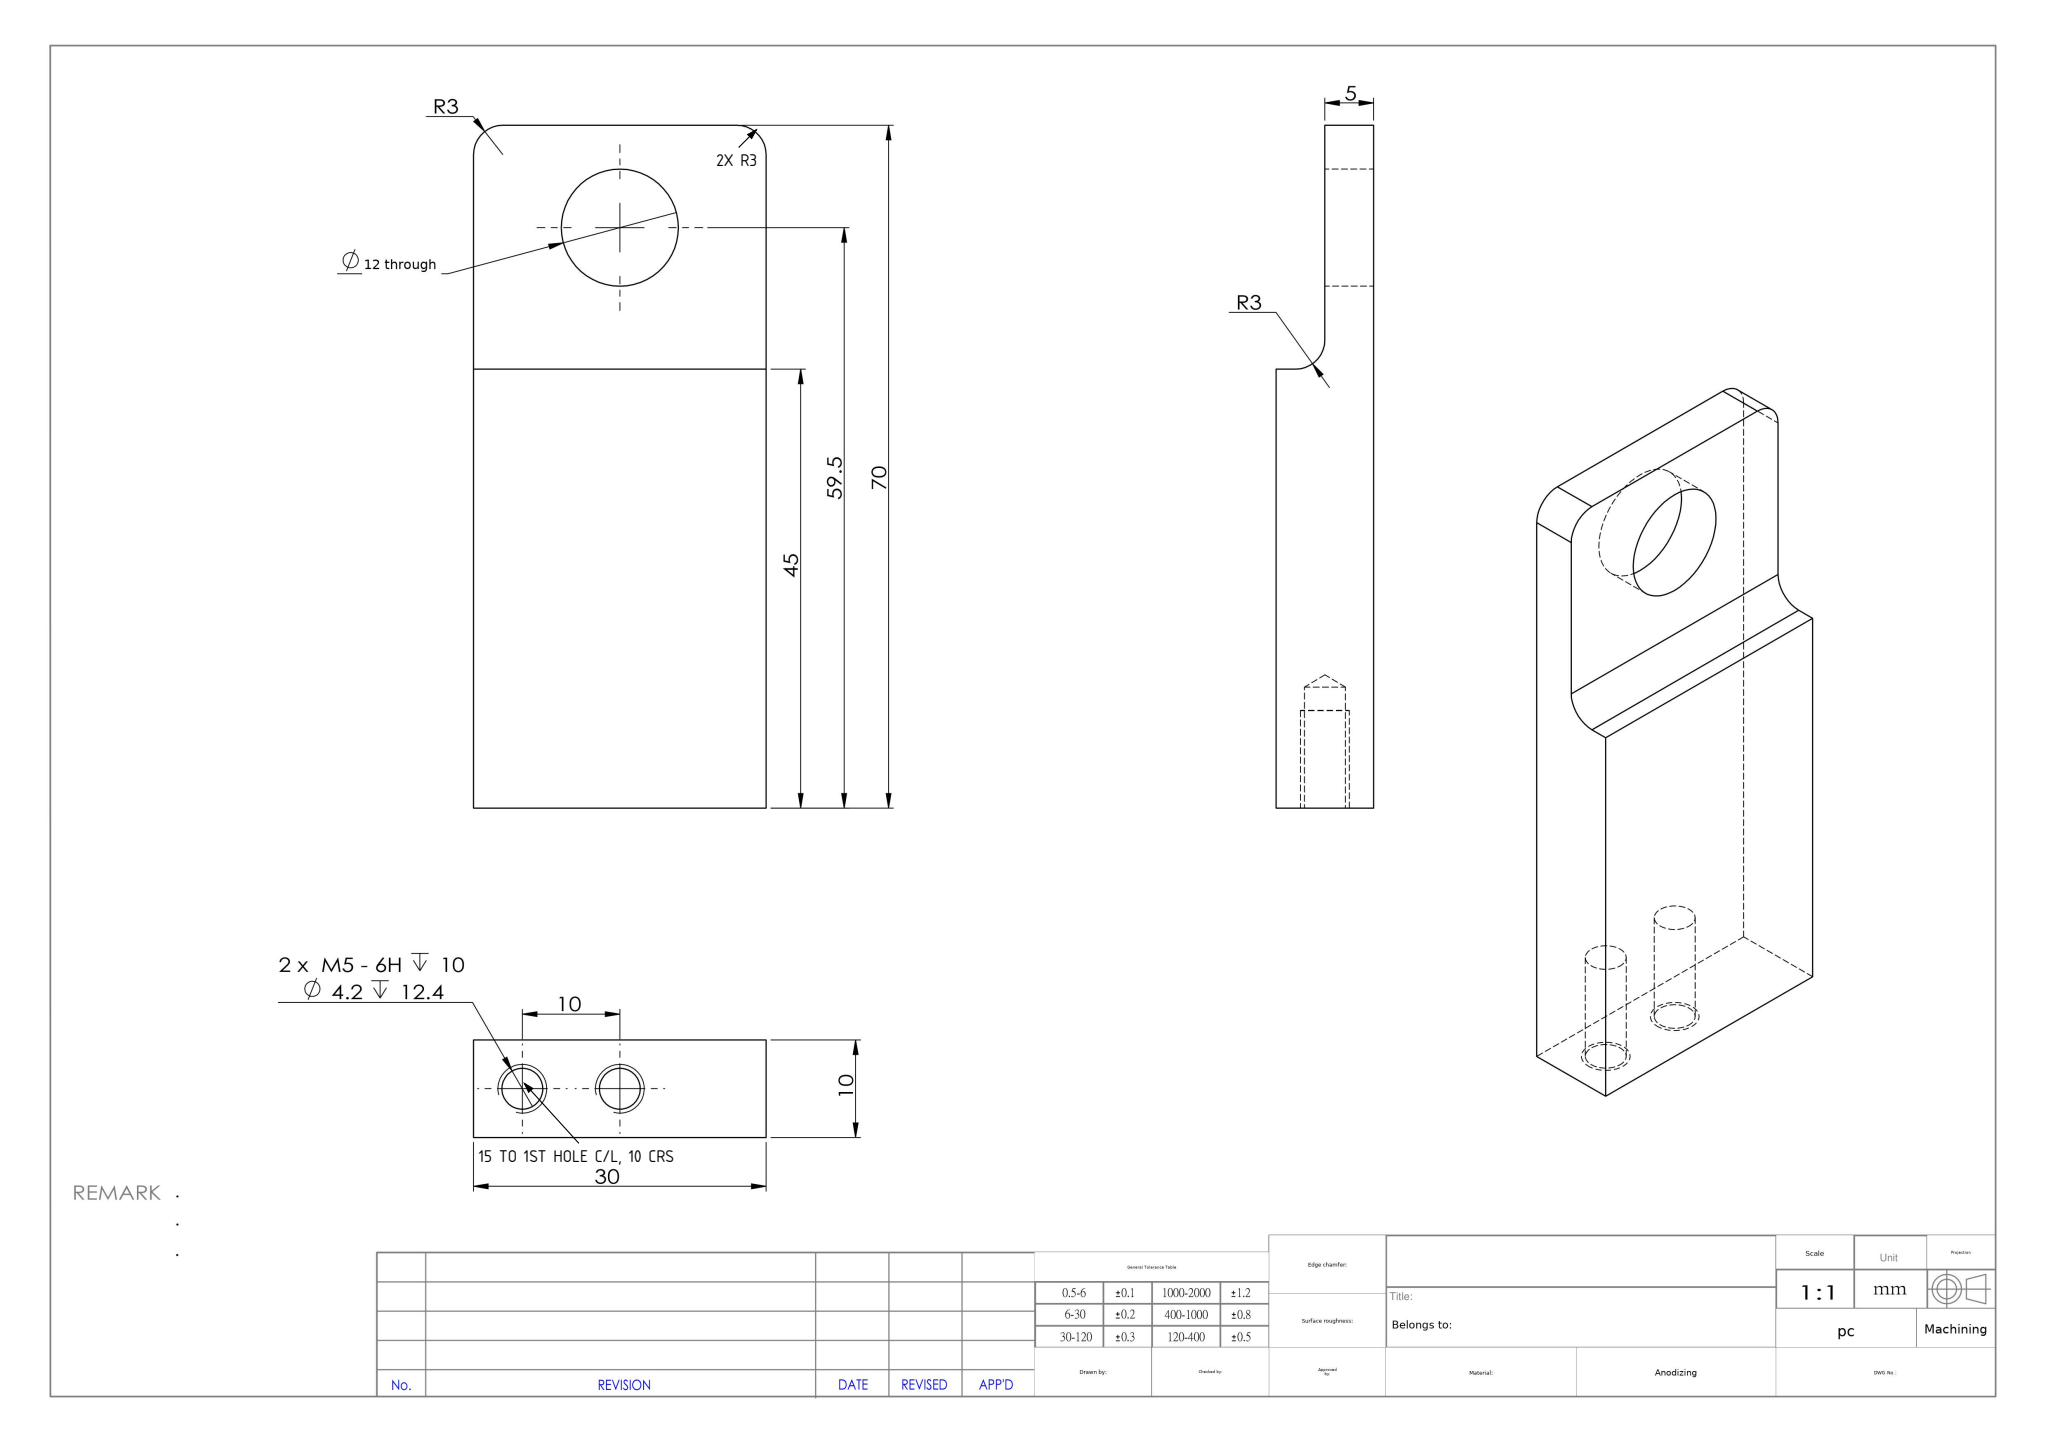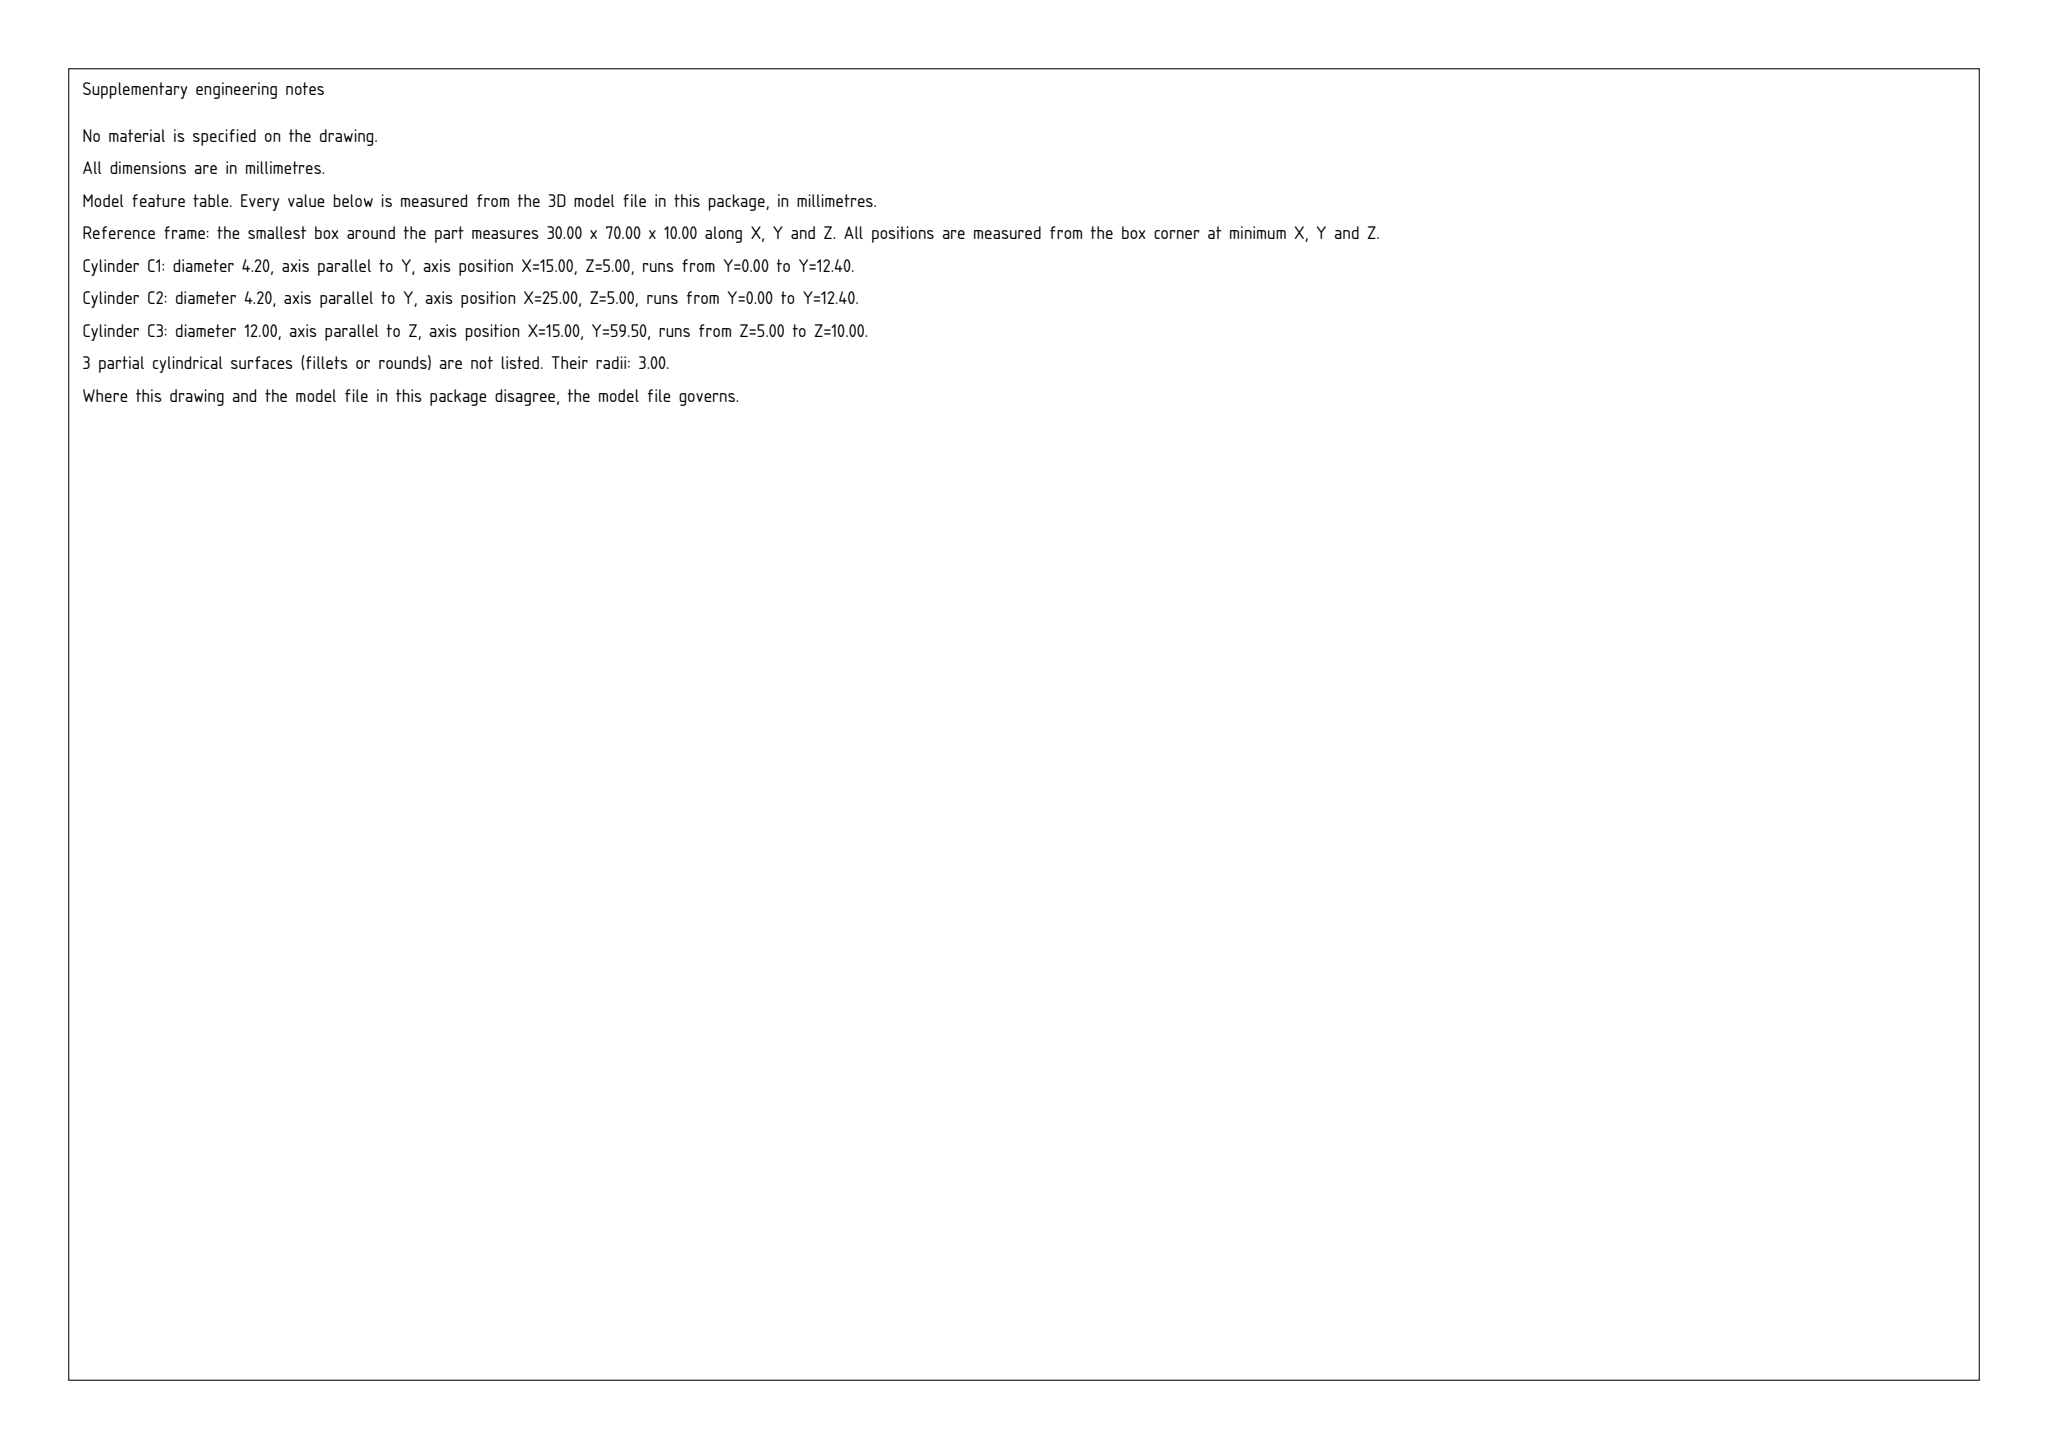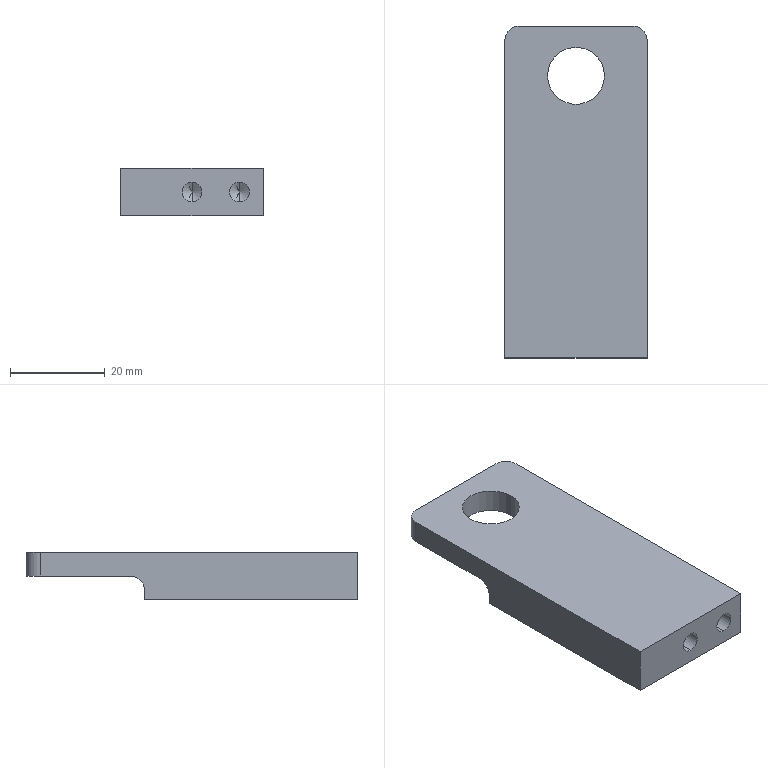Part | SolidWorks | mm | 1 solid | 21 faces | box 30 x 70 x 10 mm | volume 16368 mm3 | cylinder 9 | plane 8 | cone 4 | commonest cylinder face diameters 4.2 x4 6 x3 12 x2
Drawing notes:
2X M5 PATTERN: 15 FROM LEFT END FACE TO 1ST HOLE C/L, 10 CRS | from the solid: Ø4.2 y-axis cylinders at x=15.0 and x=25.0 in 30.0 wide bbox
TAB TOP CORNERS R3 TYP (2X) | from the solid: Ø6 z-axis corner cylinders at (3,67) and (27,67), r=3, 5 deep
build123d program:
from build123d import *

# Parameters (mm, degrees)
SKETCH1_W             = 30
SKETCH1_H             = 5
BOSS_EXTRUDE1_DEPTH   = 70
SKETCH3_W             = 30
SKETCH3_H             = 45
BOSS_EXTRUDE2_DEPTH   = 5
M5_TAPPED_HOLE1_D     = 4.2
M5_TAPPED_HOLE1_DEPTH = 12.4
M5_TAPPED_HOLE1_TIP   = 1.262
SKETCH7_R             = 6
CUT_EXTRUDE1_DEPTH    = 72.764
FILLET1_R             = 3


with BuildPart() as part:
    # Sketch1 → Boss-Extrude1 (new body)
    with BuildSketch(Plane(origin=(0, 0, 0), x_dir=(1, 0, 0), z_dir=(0, 1, 0))):
        Rectangle(SKETCH1_W, SKETCH1_H)
    extrude(amount=BOSS_EXTRUDE1_DEPTH)

    # Sketch3 → Boss-Extrude2 (add)
    with BuildSketch(Plane(origin=(0, 0, -2.5), x_dir=(-1, 0, 0), z_dir=(0, 0, -1))):
        with Locations((0, 22.5)):
            Rectangle(SKETCH3_W, SKETCH3_H)
    extrude(amount=BOSS_EXTRUDE2_DEPTH)

    # M5 Tapped Hole1
    with Locations(Plane(origin=(0, 0, 0), x_dir=(-1, 0, 0), z_dir=(0, -1, 0))):
        with Locations((0, 2.5), (-10, 2.5)):
            Hole(M5_TAPPED_HOLE1_D / 2, depth=M5_TAPPED_HOLE1_DEPTH)
            with Locations((0, 0, -(M5_TAPPED_HOLE1_DEPTH + M5_TAPPED_HOLE1_TIP / 2))):  # 118° drill point
                Cone(0, M5_TAPPED_HOLE1_D / 2, M5_TAPPED_HOLE1_TIP, mode=Mode.SUBTRACT)

    # Sketch7 → Cut-Extrude1 (cut, through all)
    with BuildSketch(Plane(origin=(0, 0, -2.5), x_dir=(-1, 0, 0), z_dir=(0, 0, -1))):
        with Locations((0, 59.5)):
            Circle(SKETCH7_R)
    extrude(amount=-CUT_EXTRUDE1_DEPTH, mode=Mode.SUBTRACT)

    # Fillet1
    fillet1_edges = [part.edges().sort_by_distance(p)[0] for p in [
        (-15, 70, 0),
        (0, 45, -2.5),
        (15, 70, 0),
    ]]
    fillet(fillet1_edges, radius=FILLET1_R)


solid = part.part
STEP:
#1=CARTESIAN_POINT('',(6.,59.5,2.5));
#2=VERTEX_POINT('',#1);
#3=CARTESIAN_POINT('',(-6.,59.5,2.5));
#4=VERTEX_POINT('',#3);
#5=CARTESIAN_POINT('',(0.,59.5,2.5));
#6=DIRECTION('',(0.,0.,-1.));
#7=DIRECTION('',(-1.,0.,0.));
#8=AXIS2_PLACEMENT_3D('',#5,#6,#7);
#9=CIRCLE('',#8,6.);
#10=EDGE_CURVE('',#2,#4,#9,.T.);
#11=ORIENTED_EDGE('',*,*,#10,.F.);
#12=CARTESIAN_POINT('',(6.,59.5,-2.5));
#13=VERTEX_POINT('',#12);
#14=CARTESIAN_POINT('',(6.,59.5,2.5));
#15=DIRECTION('',(0.,0.,-1.));
#16=VECTOR('',#15,1000.);
#17=LINE('',#14,#16);
#18=EDGE_CURVE('',#2,#13,#17,.T.);
#19=ORIENTED_EDGE('',*,*,#18,.T.);
#20=CARTESIAN_POINT('',(-6.,59.5,-2.5));
#21=VERTEX_POINT('',#20);
#22=CARTESIAN_POINT('',(0.,59.5,-2.5));
#23=DIRECTION('',(0.,0.,-1.));
#24=DIRECTION('',(-1.,0.,0.));
#25=AXIS2_PLACEMENT_3D('',#22,#23,#24);
#26=CIRCLE('',#25,6.);
#27=EDGE_CURVE('',#13,#21,#26,.T.);
#28=ORIENTED_EDGE('',*,*,#27,.T.);
#29=CARTESIAN_POINT('',(-6.,59.5,2.5));
#30=DIRECTION('',(0.,0.,-1.));
#31=VECTOR('',#30,1000.);
#32=LINE('',#29,#31);
#33=EDGE_CURVE('',#4,#21,#32,.T.);
#34=ORIENTED_EDGE('',*,*,#33,.F.);
#35=EDGE_LOOP('',(#11,#19,#28,#34));
#36=FACE_OUTER_BOUND('',#35,.T.);
#37=CARTESIAN_POINT('',(0.,59.5,2.5));
#38=DIRECTION('',(0.,0.,-1.));
#39=DIRECTION('',(-1.,0.,0.));
#40=AXIS2_PLACEMENT_3D('',#37,#38,#39);
#41=CYLINDRICAL_SURFACE('',#40,6.);
#42=ADVANCED_FACE('',(#36),#41,.F.);
#43=CARTESIAN_POINT('',(0.,12.4,-0.4));
#44=VERTEX_POINT('',#43);
#45=CARTESIAN_POINT('',(0.,12.4,-4.6));
#46=VERTEX_POINT('',#45);
#47=CARTESIAN_POINT('',(0.,12.4,-2.5));
#48=DIRECTION('',(0.,-1.,0.));
#49=DIRECTION('',(0.,0.,-1.));
#50=AXIS2_PLACEMENT_3D('',#47,#48,#49);
#51=CIRCLE('',#50,2.1);
#52=EDGE_CURVE('',#44,#46,#51,.T.);
#53=ORIENTED_EDGE('',*,*,#52,.F.);
#54=CARTESIAN_POINT('',(0.,-0.,-0.4));
#55=VERTEX_POINT('',#54);
#56=CARTESIAN_POINT('',(0.,0.,-0.4));
#57=DIRECTION('',(0.,-1.,0.));
#58=VECTOR('',#57,1000.);
#59=LINE('',#56,#58);
#60=EDGE_CURVE('',#44,#55,#59,.T.);
#61=ORIENTED_EDGE('',*,*,#60,.T.);
#62=CARTESIAN_POINT('',(0.,-0.,-4.6));
#63=VERTEX_POINT('',#62);
#64=CARTESIAN_POINT('',(0.,-0.,-2.5));
#65=DIRECTION('',(0.,-1.,0.));
#66=DIRECTION('',(0.,0.,-1.));
#67=AXIS2_PLACEMENT_3D('',#64,#65,#66);
#68=CIRCLE('',#67,2.1);
#69=EDGE_CURVE('',#55,#63,#68,.T.);
#70=ORIENTED_EDGE('',*,*,#69,.T.);
#71=CARTESIAN_POINT('',(0.,0.,-4.6));
#72=DIRECTION('',(0.,-1.,0.));
#73=VECTOR('',#72,1000.);
#74=LINE('',#71,#73);
#75=EDGE_CURVE('',#46,#63,#74,.T.);
#76=ORIENTED_EDGE('',*,*,#75,.F.);
#77=EDGE_LOOP('',(#53,#61,#70,#76));
#78=FACE_OUTER_BOUND('',#77,.T.);
#79=CARTESIAN_POINT('',(0.,0.,-2.5));
#80=DIRECTION('',(0.,-1.,0.));
#81=DIRECTION('',(0.,0.,-1.));
#82=AXIS2_PLACEMENT_3D('',#79,#80,#81);
#83=CYLINDRICAL_SURFACE('',#82,2.1);
#84=ADVANCED_FACE('',(#78),#83,.F.);
#85=CARTESIAN_POINT('',(-0.,13.662,-2.5));
#86=VERTEX_POINT('',#85);
#87=CARTESIAN_POINT('',(0.,12.4,-4.6));
#88=DIRECTION('',(0.,-0.515,-0.8572));
#89=VECTOR('',#88,1000.);
#90=LINE('',#87,#89);
#91=EDGE_CURVE('',#86,#46,#90,.T.);
#92=ORIENTED_EDGE('',*,*,#91,.F.);
#93=CARTESIAN_POINT('',(0.,12.4,-0.4));
#94=DIRECTION('',(0.,-0.515,0.8572));
#95=VECTOR('',#94,1000.);
#96=LINE('',#93,#95);
#97=EDGE_CURVE('',#86,#44,#96,.T.);
#98=ORIENTED_EDGE('',*,*,#97,.T.);
#99=ORIENTED_EDGE('',*,*,#52,.T.);
#100=EDGE_LOOP('',(#92,#98,#99));
#101=FACE_OUTER_BOUND('',#100,.T.);
#102=CARTESIAN_POINT('',(0.,12.4,-2.5));
#103=DIRECTION('',(0.,-1.,0.));
#104=DIRECTION('',(0.,0.,-1.));
#105=AXIS2_PLACEMENT_3D('',#102,#103,#104);
#106=CONICAL_SURFACE('',#105,2.1,1.03);
#107=ADVANCED_FACE('',(#101),#106,.F.);
#108=CARTESIAN_POINT('',(10.,12.4,-0.4));
#109=VERTEX_POINT('',#108);
#110=CARTESIAN_POINT('',(10.,12.4,-4.6));
#111=VERTEX_POINT('',#110);
#112=CARTESIAN_POINT('',(10.,12.4,-2.5));
#113=DIRECTION('',(0.,-1.,0.));
#114=DIRECTION('',(0.,0.,-1.));
#115=AXIS2_PLACEMENT_3D('',#112,#113,#114);
#116=CIRCLE('',#115,2.1);
#117=EDGE_CURVE('',#109,#111,#116,.T.);
#118=ORIENTED_EDGE('',*,*,#117,.F.);
#119=CARTESIAN_POINT('',(10.,-0.,-0.4));
#120=VERTEX_POINT('',#119);
#121=CARTESIAN_POINT('',(10.,0.,-0.4));
#122=DIRECTION('',(0.,-1.,0.));
#123=VECTOR('',#122,1000.);
#124=LINE('',#121,#123);
#125=EDGE_CURVE('',#109,#120,#124,.T.);
#126=ORIENTED_EDGE('',*,*,#125,.T.);
#127=CARTESIAN_POINT('',(10.,-0.,-4.6));
#128=VERTEX_POINT('',#127);
#129=CARTESIAN_POINT('',(10.,-0.,-2.5));
#130=DIRECTION('',(0.,-1.,0.));
#131=DIRECTION('',(0.,0.,-1.));
#132=AXIS2_PLACEMENT_3D('',#129,#130,#131);
#133=CIRCLE('',#132,2.1);
#134=EDGE_CURVE('',#120,#128,#133,.T.);
#135=ORIENTED_EDGE('',*,*,#134,.T.);
#136=CARTESIAN_POINT('',(10.,0.,-4.6));
#137=DIRECTION('',(0.,-1.,0.));
#138=VECTOR('',#137,1000.);
#139=LINE('',#136,#138);
#140=EDGE_CURVE('',#111,#128,#139,.T.);
#141=ORIENTED_EDGE('',*,*,#140,.F.);
#142=EDGE_LOOP('',(#118,#126,#135,#141));
#143=FACE_OUTER_BOUND('',#142,.T.);
#144=CARTESIAN_POINT('',(10.,0.,-2.5));
#145=DIRECTION('',(0.,-1.,0.));
#146=DIRECTION('',(0.,0.,-1.));
#147=AXIS2_PLACEMENT_3D('',#144,#145,#146);
#148=CYLINDRICAL_SURFACE('',#147,2.1);
#149=ADVANCED_FACE('',(#143),#148,.F.);
#150=CARTESIAN_POINT('',(10.,13.662,-2.5));
#151=VERTEX_POINT('',#150);
#152=CARTESIAN_POINT('',(10.,12.4,-4.6));
#153=DIRECTION('',(0.,-0.515,-0.8572));
#154=VECTOR('',#153,1000.);
#155=LINE('',#152,#154);
#156=EDGE_CURVE('',#151,#111,#155,.T.);
#157=ORIENTED_EDGE('',*,*,#156,.F.);
#158=CARTESIAN_POINT('',(10.,12.4,-0.4));
#159=DIRECTION('',(0.,-0.515,0.8572));
#160=VECTOR('',#159,1000.);
#161=LINE('',#158,#160);
#162=EDGE_CURVE('',#151,#109,#161,.T.);
#163=ORIENTED_EDGE('',*,*,#162,.T.);
#164=ORIENTED_EDGE('',*,*,#117,.T.);
#165=EDGE_LOOP('',(#157,#163,#164));
#166=FACE_OUTER_BOUND('',#165,.T.);
#167=CARTESIAN_POINT('',(10.,12.4,-2.5));
#168=DIRECTION('',(0.,-1.,0.));
#169=DIRECTION('',(0.,0.,-1.));
#170=AXIS2_PLACEMENT_3D('',#167,#168,#169);
#171=CONICAL_SURFACE('',#170,2.1,1.03);
#172=ADVANCED_FACE('',(#166),#171,.F.);
#173=CARTESIAN_POINT('',(0.,59.5,-2.5));
#174=DIRECTION('',(0.,0.,-1.));
#175=DIRECTION('',(-1.,0.,0.));
#176=AXIS2_PLACEMENT_3D('',#173,#174,#175);
#177=CIRCLE('',#176,6.);
#178=EDGE_CURVE('',#21,#13,#177,.T.);
#179=ORIENTED_EDGE('',*,*,#178,.F.);
#180=ORIENTED_EDGE('',*,*,#27,.F.);
#181=EDGE_LOOP('',(#179,#180));
#182=FACE_BOUND('',#181,.T.);
#183=CARTESIAN_POINT('',(15.,67.,-2.5));
#184=VERTEX_POINT('',#183);
#185=CARTESIAN_POINT('',(15.,48.,-2.5));
#186=VERTEX_POINT('',#185);
#187=CARTESIAN_POINT('',(15.,70.,-2.5));
#188=DIRECTION('',(0.,-1.,0.));
#189=VECTOR('',#188,1000.);
#190=LINE('',#187,#189);
#191=EDGE_CURVE('',#184,#186,#190,.T.);
#192=ORIENTED_EDGE('',*,*,#191,.T.);
#193=CARTESIAN_POINT('',(-15.,48.,-2.5));
#194=VERTEX_POINT('',#193);
#195=CARTESIAN_POINT('',(-15.,48.,-2.5));
#196=DIRECTION('',(-1.,0.,0.));
#197=VECTOR('',#196,1000.);
#198=LINE('',#195,#197);
#199=EDGE_CURVE('',#186,#194,#198,.T.);
#200=ORIENTED_EDGE('',*,*,#199,.T.);
#201=CARTESIAN_POINT('',(-15.,67.,-2.5));
#202=VERTEX_POINT('',#201);
#203=CARTESIAN_POINT('',(-15.,70.,-2.5));
#204=DIRECTION('',(0.,-1.,0.));
#205=VECTOR('',#204,1000.);
#206=LINE('',#203,#205);
#207=EDGE_CURVE('',#202,#194,#206,.T.);
#208=ORIENTED_EDGE('',*,*,#207,.F.);
#209=CARTESIAN_POINT('',(-12.,70.,-2.5));
#210=VERTEX_POINT('',#209);
#211=CARTESIAN_POINT('',(-12.,67.,-2.5));
#212=DIRECTION('',(0.,0.,-1.));
#213=DIRECTION('',(1.,0.,0.));
#214=AXIS2_PLACEMENT_3D('',#211,#212,#213);
#215=CIRCLE('',#214,3.);
#216=EDGE_CURVE('',#202,#210,#215,.T.);
#217=ORIENTED_EDGE('',*,*,#216,.T.);
#218=CARTESIAN_POINT('',(12.,70.,-2.5));
#219=VERTEX_POINT('',#218);
#220=CARTESIAN_POINT('',(-15.,70.,-2.5));
#221=DIRECTION('',(-1.,0.,0.));
#222=VECTOR('',#221,1000.);
#223=LINE('',#220,#222);
#224=EDGE_CURVE('',#219,#210,#223,.T.);
#225=ORIENTED_EDGE('',*,*,#224,.F.);
#226=CARTESIAN_POINT('',(12.,67.,-2.5));
#227=DIRECTION('',(0.,0.,-1.));
#228=DIRECTION('',(1.,0.,0.));
#229=AXIS2_PLACEMENT_3D('',#226,#227,#228);
#230=CIRCLE('',#229,3.);
#231=EDGE_CURVE('',#219,#184,#230,.T.);
#232=ORIENTED_EDGE('',*,*,#231,.T.);
#233=EDGE_LOOP('',(#192,#200,#208,#217,#225,#232));
#234=FACE_OUTER_BOUND('',#233,.T.);
#235=CARTESIAN_POINT('',(-15.,70.,-2.5));
#236=DIRECTION('',(0.,0.,1.));
#237=DIRECTION('',(1.,0.,0.));
#238=AXIS2_PLACEMENT_3D('',#235,#236,#237);
#239=PLANE('',#238);
#240=ADVANCED_FACE('',(#182,#234),#239,.F.);
#241=ORIENTED_EDGE('',*,*,#191,.F.);
#242=CARTESIAN_POINT('',(15.,67.,2.5));
#243=VERTEX_POINT('',#242);
#244=CARTESIAN_POINT('',(15.,67.,2.5));
#245=DIRECTION('',(0.,0.,1.));
#246=VECTOR('',#245,1000.);
#247=LINE('',#244,#246);
#248=EDGE_CURVE('',#184,#243,#247,.T.);
#249=ORIENTED_EDGE('',*,*,#248,.T.);
#250=CARTESIAN_POINT('',(15.,0.,2.5));
#251=VERTEX_POINT('',#250);
#252=CARTESIAN_POINT('',(15.,70.,2.5));
#253=DIRECTION('',(0.,-1.,0.));
#254=VECTOR('',#253,1000.);
#255=LINE('',#252,#254);
#256=EDGE_CURVE('',#243,#251,#255,.T.);
#257=ORIENTED_EDGE('',*,*,#256,.T.);
#258=CARTESIAN_POINT('',(15.,0.,-7.5));
#259=VERTEX_POINT('',#258);
#260=CARTESIAN_POINT('',(15.,0.,2.5));
#261=DIRECTION('',(0.,0.,-1.));
#262=VECTOR('',#261,1000.);
#263=LINE('',#260,#262);
#264=EDGE_CURVE('',#251,#259,#263,.T.);
#265=ORIENTED_EDGE('',*,*,#264,.T.);
#266=CARTESIAN_POINT('',(15.,45.,-7.5));
#267=VERTEX_POINT('',#266);
#268=CARTESIAN_POINT('',(15.,0.,-7.5));
#269=DIRECTION('',(0.,-1.,0.));
#270=VECTOR('',#269,1000.);
#271=LINE('',#268,#270);
#272=EDGE_CURVE('',#267,#259,#271,.T.);
#273=ORIENTED_EDGE('',*,*,#272,.F.);
#274=CARTESIAN_POINT('',(15.,45.,-5.5));
#275=VERTEX_POINT('',#274);
#276=CARTESIAN_POINT('',(15.,45.,-7.5));
#277=DIRECTION('',(0.,0.,1.));
#278=VECTOR('',#277,1000.);
#279=LINE('',#276,#278);
#280=EDGE_CURVE('',#267,#275,#279,.T.);
#281=ORIENTED_EDGE('',*,*,#280,.T.);
#282=CARTESIAN_POINT('',(15.,48.,-5.5));
#283=DIRECTION('',(-1.,0.,0.));
#284=DIRECTION('',(0.,0.,1.));
#285=AXIS2_PLACEMENT_3D('',#282,#283,#284);
#286=CIRCLE('',#285,3.);
#287=EDGE_CURVE('',#275,#186,#286,.T.);
#288=ORIENTED_EDGE('',*,*,#287,.T.);
#289=EDGE_LOOP('',(#241,#249,#257,#265,#273,#281,#288));
#290=FACE_OUTER_BOUND('',#289,.T.);
#291=CARTESIAN_POINT('',(15.,70.,2.5));
#292=DIRECTION('',(-1.,0.,0.));
#293=DIRECTION('',(0.,0.,1.));
#294=AXIS2_PLACEMENT_3D('',#291,#292,#293);
#295=PLANE('',#294);
#296=ADVANCED_FACE('',(#290),#295,.F.);
#297=CARTESIAN_POINT('',(-15.,67.,2.5));
#298=VERTEX_POINT('',#297);
#299=CARTESIAN_POINT('',(-15.,0.,2.5));
#300=VERTEX_POINT('',#299);
#301=CARTESIAN_POINT('',(-15.,70.,2.5));
#302=DIRECTION('',(0.,-1.,0.));
#303=VECTOR('',#302,1000.);
#304=LINE('',#301,#303);
#305=EDGE_CURVE('',#298,#300,#304,.T.);
#306=ORIENTED_EDGE('',*,*,#305,.F.);
#307=CARTESIAN_POINT('',(-15.,67.,2.5));
#308=DIRECTION('',(0.,0.,-1.));
#309=VECTOR('',#308,1000.);
#310=LINE('',#307,#309);
#311=EDGE_CURVE('',#298,#202,#310,.T.);
#312=ORIENTED_EDGE('',*,*,#311,.T.);
#313=ORIENTED_EDGE('',*,*,#207,.T.);
#314=CARTESIAN_POINT('',(-15.,45.,-5.5));
#315=VERTEX_POINT('',#314);
#316=CARTESIAN_POINT('',(-15.,48.,-5.5));
#317=DIRECTION('',(1.,0.,0.));
#318=DIRECTION('',(0.,0.,-1.));
#319=AXIS2_PLACEMENT_3D('',#316,#317,#318);
#320=CIRCLE('',#319,3.);
#321=EDGE_CURVE('',#194,#315,#320,.T.);
#322=ORIENTED_EDGE('',*,*,#321,.T.);
#323=CARTESIAN_POINT('',(-15.,45.,-7.5));
#324=VERTEX_POINT('',#323);
#325=CARTESIAN_POINT('',(-15.,45.,-7.5));
#326=DIRECTION('',(0.,0.,1.));
#327=VECTOR('',#326,1000.);
#328=LINE('',#325,#327);
#329=EDGE_CURVE('',#324,#315,#328,.T.);
#330=ORIENTED_EDGE('',*,*,#329,.F.);
#331=CARTESIAN_POINT('',(-15.,0.,-7.5));
#332=VERTEX_POINT('',#331);
#333=CARTESIAN_POINT('',(-15.,0.,-7.5));
#334=DIRECTION('',(0.,1.,0.));
#335=VECTOR('',#334,1000.);
#336=LINE('',#333,#335);
#337=EDGE_CURVE('',#332,#324,#336,.T.);
#338=ORIENTED_EDGE('',*,*,#337,.F.);
#339=CARTESIAN_POINT('',(-15.,0.,2.5));
#340=DIRECTION('',(0.,0.,1.));
#341=VECTOR('',#340,1000.);
#342=LINE('',#339,#341);
#343=EDGE_CURVE('',#332,#300,#342,.T.);
#344=ORIENTED_EDGE('',*,*,#343,.T.);
#345=EDGE_LOOP('',(#306,#312,#313,#322,#330,#338,#344));
#346=FACE_OUTER_BOUND('',#345,.T.);
#347=CARTESIAN_POINT('',(-15.,70.,2.5));
#348=DIRECTION('',(1.,0.,0.));
#349=DIRECTION('',(0.,0.,-1.));
#350=AXIS2_PLACEMENT_3D('',#347,#348,#349);
#351=PLANE('',#350);
#352=ADVANCED_FACE('',(#346),#351,.F.);
#353=CARTESIAN_POINT('',(0.,59.5,2.5));
#354=DIRECTION('',(0.,0.,-1.));
#355=DIRECTION('',(-1.,0.,0.));
#356=AXIS2_PLACEMENT_3D('',#353,#354,#355);
#357=CIRCLE('',#356,6.);
#358=EDGE_CURVE('',#4,#2,#357,.T.);
#359=ORIENTED_EDGE('',*,*,#358,.T.);
#360=ORIENTED_EDGE('',*,*,#10,.T.);
#361=EDGE_LOOP('',(#359,#360));
#362=FACE_BOUND('',#361,.T.);
#363=CARTESIAN_POINT('',(-12.,70.,2.5));
#364=VERTEX_POINT('',#363);
#365=CARTESIAN_POINT('',(12.,70.,2.5));
#366=VERTEX_POINT('',#365);
#367=CARTESIAN_POINT('',(-15.,70.,2.5));
#368=DIRECTION('',(1.,0.,0.));
#369=VECTOR('',#368,1000.);
#370=LINE('',#367,#369);
#371=EDGE_CURVE('',#364,#366,#370,.T.);
#372=ORIENTED_EDGE('',*,*,#371,.F.);
#373=CARTESIAN_POINT('',(-12.,67.,2.5));
#374=DIRECTION('',(0.,0.,1.));
#375=DIRECTION('',(-1.,0.,0.));
#376=AXIS2_PLACEMENT_3D('',#373,#374,#375);
#377=CIRCLE('',#376,3.);
#378=EDGE_CURVE('',#364,#298,#377,.T.);
#379=ORIENTED_EDGE('',*,*,#378,.T.);
#380=ORIENTED_EDGE('',*,*,#305,.T.);
#381=CARTESIAN_POINT('',(-15.,0.,2.5));
#382=DIRECTION('',(1.,0.,0.));
#383=VECTOR('',#382,1000.);
#384=LINE('',#381,#383);
#385=EDGE_CURVE('',#300,#251,#384,.T.);
#386=ORIENTED_EDGE('',*,*,#385,.T.);
#387=ORIENTED_EDGE('',*,*,#256,.F.);
#388=CARTESIAN_POINT('',(12.,67.,2.5));
#389=DIRECTION('',(0.,0.,1.));
#390=DIRECTION('',(-1.,0.,0.));
#391=AXIS2_PLACEMENT_3D('',#388,#389,#390);
#392=CIRCLE('',#391,3.);
#393=EDGE_CURVE('',#243,#366,#392,.T.);
#394=ORIENTED_EDGE('',*,*,#393,.T.);
#395=EDGE_LOOP('',(#372,#379,#380,#386,#387,#394));
#396=FACE_OUTER_BOUND('',#395,.T.);
#397=CARTESIAN_POINT('',(-15.,70.,2.5));
#398=DIRECTION('',(0.,0.,-1.));
#399=DIRECTION('',(-1.,0.,0.));
#400=AXIS2_PLACEMENT_3D('',#397,#398,#399);
#401=PLANE('',#400);
#402=ADVANCED_FACE('',(#362,#396),#401,.F.);
#403=ORIENTED_EDGE('',*,*,#224,.T.);
#404=CARTESIAN_POINT('',(-12.,70.,0.));
#405=DIRECTION('',(0.,0.,1.));
#406=VECTOR('',#405,1000.);
#407=LINE('',#404,#406);
#408=EDGE_CURVE('',#210,#364,#407,.T.);
#409=ORIENTED_EDGE('',*,*,#408,.T.);
#410=ORIENTED_EDGE('',*,*,#371,.T.);
#411=CARTESIAN_POINT('',(12.,70.,0.));
#412=DIRECTION('',(0.,0.,-1.));
#413=VECTOR('',#412,1000.);
#414=LINE('',#411,#413);
#415=EDGE_CURVE('',#366,#219,#414,.T.);
#416=ORIENTED_EDGE('',*,*,#415,.T.);
#417=EDGE_LOOP('',(#403,#409,#410,#416));
#418=FACE_OUTER_BOUND('',#417,.T.);
#419=CARTESIAN_POINT('',(0.,70.,0.));
#420=DIRECTION('',(0.,-1.,0.));
#421=DIRECTION('',(0.,0.,-1.));
#422=AXIS2_PLACEMENT_3D('',#419,#420,#421);
#423=PLANE('',#422);
#424=ADVANCED_FACE('',(#418),#423,.F.);
#425=CARTESIAN_POINT('',(0.,-0.,-2.5));
#426=DIRECTION('',(0.,-1.,0.));
#427=DIRECTION('',(0.,0.,-1.));
#428=AXIS2_PLACEMENT_3D('',#425,#426,#427);
#429=CIRCLE('',#428,2.1);
#430=EDGE_CURVE('',#63,#55,#429,.T.);
#431=ORIENTED_EDGE('',*,*,#430,.F.);
#432=ORIENTED_EDGE('',*,*,#69,.F.);
#433=EDGE_LOOP('',(#431,#432));
#434=FACE_BOUND('',#433,.T.);
#435=CARTESIAN_POINT('',(10.,-0.,-2.5));
#436=DIRECTION('',(0.,-1.,0.));
#437=DIRECTION('',(0.,0.,-1.));
#438=AXIS2_PLACEMENT_3D('',#435,#436,#437);
#439=CIRCLE('',#438,2.1);
#440=EDGE_CURVE('',#128,#120,#439,.T.);
#441=ORIENTED_EDGE('',*,*,#440,.F.);
#442=ORIENTED_EDGE('',*,*,#134,.F.);
#443=EDGE_LOOP('',(#441,#442));
#444=FACE_BOUND('',#443,.T.);
#445=ORIENTED_EDGE('',*,*,#264,.F.);
#446=ORIENTED_EDGE('',*,*,#385,.F.);
#447=ORIENTED_EDGE('',*,*,#343,.F.);
#448=CARTESIAN_POINT('',(15.,0.,-7.5));
#449=DIRECTION('',(-1.,0.,0.));
#450=VECTOR('',#449,1000.);
#451=LINE('',#448,#450);
#452=EDGE_CURVE('',#259,#332,#451,.T.);
#453=ORIENTED_EDGE('',*,*,#452,.F.);
#454=EDGE_LOOP('',(#445,#446,#447,#453));
#455=FACE_OUTER_BOUND('',#454,.T.);
#456=CARTESIAN_POINT('',(0.,0.,0.));
#457=DIRECTION('',(0.,-1.,0.));
#458=DIRECTION('',(0.,0.,-1.));
#459=AXIS2_PLACEMENT_3D('',#456,#457,#458);
#460=PLANE('',#459);
#461=ADVANCED_FACE('',(#434,#444,#455),#460,.T.);
#462=ORIENTED_EDGE('',*,*,#329,.T.);
#463=CARTESIAN_POINT('',(15.,45.,-5.5));
#464=DIRECTION('',(1.,0.,0.));
#465=VECTOR('',#464,1000.);
#466=LINE('',#463,#465);
#467=EDGE_CURVE('',#315,#275,#466,.T.);
#468=ORIENTED_EDGE('',*,*,#467,.T.);
#469=ORIENTED_EDGE('',*,*,#280,.F.);
#470=CARTESIAN_POINT('',(15.,45.,-7.5));
#471=DIRECTION('',(1.,0.,0.));
#472=VECTOR('',#471,1000.);
#473=LINE('',#470,#472);
#474=EDGE_CURVE('',#324,#267,#473,.T.);
#475=ORIENTED_EDGE('',*,*,#474,.F.);
#476=EDGE_LOOP('',(#462,#468,#469,#475));
#477=FACE_OUTER_BOUND('',#476,.T.);
#478=CARTESIAN_POINT('',(15.,45.,-7.5));
#479=DIRECTION('',(0.,-1.,0.));
#480=DIRECTION('',(0.,0.,-1.));
#481=AXIS2_PLACEMENT_3D('',#478,#479,#480);
#482=PLANE('',#481);
#483=ADVANCED_FACE('',(#477),#482,.F.);
#484=ORIENTED_EDGE('',*,*,#272,.T.);
#485=ORIENTED_EDGE('',*,*,#452,.T.);
#486=ORIENTED_EDGE('',*,*,#337,.T.);
#487=ORIENTED_EDGE('',*,*,#474,.T.);
#488=EDGE_LOOP('',(#484,#485,#486,#487));
#489=FACE_OUTER_BOUND('',#488,.T.);
#490=CARTESIAN_POINT('',(0.,0.,-7.5));
#491=DIRECTION('',(0.,0.,1.));
#492=DIRECTION('',(1.,0.,0.));
#493=AXIS2_PLACEMENT_3D('',#490,#491,#492);
#494=PLANE('',#493);
#495=ADVANCED_FACE('',(#489),#494,.F.);
#496=ORIENTED_EDGE('',*,*,#162,.F.);
#497=ORIENTED_EDGE('',*,*,#156,.T.);
#498=CARTESIAN_POINT('',(10.,12.4,-2.5));
#499=DIRECTION('',(0.,-1.,0.));
#500=DIRECTION('',(0.,0.,-1.));
#501=AXIS2_PLACEMENT_3D('',#498,#499,#500);
#502=CIRCLE('',#501,2.1);
#503=EDGE_CURVE('',#111,#109,#502,.T.);
#504=ORIENTED_EDGE('',*,*,#503,.T.);
#505=EDGE_LOOP('',(#496,#497,#504));
#506=FACE_OUTER_BOUND('',#505,.T.);
#507=CARTESIAN_POINT('',(10.,12.4,-2.5));
#508=DIRECTION('',(0.,-1.,0.));
#509=DIRECTION('',(0.,0.,-1.));
#510=AXIS2_PLACEMENT_3D('',#507,#508,#509);
#511=CONICAL_SURFACE('',#510,2.1,1.03);
#512=ADVANCED_FACE('',(#506),#511,.F.);
#513=ORIENTED_EDGE('',*,*,#125,.F.);
#514=ORIENTED_EDGE('',*,*,#503,.F.);
#515=ORIENTED_EDGE('',*,*,#140,.T.);
#516=ORIENTED_EDGE('',*,*,#440,.T.);
#517=EDGE_LOOP('',(#513,#514,#515,#516));
#518=FACE_OUTER_BOUND('',#517,.T.);
#519=CARTESIAN_POINT('',(10.,0.,-2.5));
#520=DIRECTION('',(0.,-1.,0.));
#521=DIRECTION('',(0.,0.,-1.));
#522=AXIS2_PLACEMENT_3D('',#519,#520,#521);
#523=CYLINDRICAL_SURFACE('',#522,2.1);
#524=ADVANCED_FACE('',(#518),#523,.F.);
#525=ORIENTED_EDGE('',*,*,#97,.F.);
#526=ORIENTED_EDGE('',*,*,#91,.T.);
#527=CARTESIAN_POINT('',(0.,12.4,-2.5));
#528=DIRECTION('',(0.,-1.,0.));
#529=DIRECTION('',(0.,0.,-1.));
#530=AXIS2_PLACEMENT_3D('',#527,#528,#529);
#531=CIRCLE('',#530,2.1);
#532=EDGE_CURVE('',#46,#44,#531,.T.);
#533=ORIENTED_EDGE('',*,*,#532,.T.);
#534=EDGE_LOOP('',(#525,#526,#533));
#535=FACE_OUTER_BOUND('',#534,.T.);
#536=CARTESIAN_POINT('',(0.,12.4,-2.5));
#537=DIRECTION('',(0.,-1.,0.));
#538=DIRECTION('',(0.,0.,-1.));
#539=AXIS2_PLACEMENT_3D('',#536,#537,#538);
#540=CONICAL_SURFACE('',#539,2.1,1.03);
#541=ADVANCED_FACE('',(#535),#540,.F.);
#542=ORIENTED_EDGE('',*,*,#60,.F.);
#543=ORIENTED_EDGE('',*,*,#532,.F.);
#544=ORIENTED_EDGE('',*,*,#75,.T.);
#545=ORIENTED_EDGE('',*,*,#430,.T.);
#546=EDGE_LOOP('',(#542,#543,#544,#545));
#547=FACE_OUTER_BOUND('',#546,.T.);
#548=CARTESIAN_POINT('',(0.,0.,-2.5));
#549=DIRECTION('',(0.,-1.,0.));
#550=DIRECTION('',(0.,0.,-1.));
#551=AXIS2_PLACEMENT_3D('',#548,#549,#550);
#552=CYLINDRICAL_SURFACE('',#551,2.1);
#553=ADVANCED_FACE('',(#547),#552,.F.);
#554=ORIENTED_EDGE('',*,*,#18,.F.);
#555=ORIENTED_EDGE('',*,*,#358,.F.);
#556=ORIENTED_EDGE('',*,*,#33,.T.);
#557=ORIENTED_EDGE('',*,*,#178,.T.);
#558=EDGE_LOOP('',(#554,#555,#556,#557));
#559=FACE_OUTER_BOUND('',#558,.T.);
#560=CARTESIAN_POINT('',(0.,59.5,2.5));
#561=DIRECTION('',(0.,0.,-1.));
#562=DIRECTION('',(-1.,0.,0.));
#563=AXIS2_PLACEMENT_3D('',#560,#561,#562);
#564=CYLINDRICAL_SURFACE('',#563,6.);
#565=ADVANCED_FACE('',(#559),#564,.F.);
#566=ORIENTED_EDGE('',*,*,#321,.F.);
#567=ORIENTED_EDGE('',*,*,#199,.F.);
#568=ORIENTED_EDGE('',*,*,#287,.F.);
#569=ORIENTED_EDGE('',*,*,#467,.F.);
#570=EDGE_LOOP('',(#566,#567,#568,#569));
#571=FACE_OUTER_BOUND('',#570,.T.);
#572=CARTESIAN_POINT('',(15.,48.,-5.5));
#573=DIRECTION('',(-1.,0.,0.));
#574=DIRECTION('',(0.,0.,1.));
#575=AXIS2_PLACEMENT_3D('',#572,#573,#574);
#576=CYLINDRICAL_SURFACE('',#575,3.);
#577=ADVANCED_FACE('',(#571),#576,.F.);
#578=ORIENTED_EDGE('',*,*,#216,.F.);
#579=ORIENTED_EDGE('',*,*,#311,.F.);
#580=ORIENTED_EDGE('',*,*,#378,.F.);
#581=ORIENTED_EDGE('',*,*,#408,.F.);
#582=EDGE_LOOP('',(#578,#579,#580,#581));
#583=FACE_OUTER_BOUND('',#582,.T.);
#584=CARTESIAN_POINT('',(-12.,67.,0.));
#585=DIRECTION('',(0.,0.,1.));
#586=DIRECTION('',(1.,0.,0.));
#587=AXIS2_PLACEMENT_3D('',#584,#585,#586);
#588=CYLINDRICAL_SURFACE('',#587,3.);
#589=ADVANCED_FACE('',(#583),#588,.T.);
#590=ORIENTED_EDGE('',*,*,#393,.F.);
#591=ORIENTED_EDGE('',*,*,#248,.F.);
#592=ORIENTED_EDGE('',*,*,#231,.F.);
#593=ORIENTED_EDGE('',*,*,#415,.F.);
#594=EDGE_LOOP('',(#590,#591,#592,#593));
#595=FACE_OUTER_BOUND('',#594,.T.);
#596=CARTESIAN_POINT('',(12.,67.,0.));
#597=DIRECTION('',(0.,0.,-1.));
#598=DIRECTION('',(-1.,0.,0.));
#599=AXIS2_PLACEMENT_3D('',#596,#597,#598);
#600=CYLINDRICAL_SURFACE('',#599,3.);
#601=ADVANCED_FACE('',(#595),#600,.T.);
#602=CLOSED_SHELL('',(#42,#84,#107,#149,#172,#240,#296,#352,#402,#424,#461,#483,#495,#512,#524,#541,#553,#565,#577,#589,#601));
#603=MANIFOLD_SOLID_BREP('',#602);
#604=CARTESIAN_POINT('',(0.,0.,0.));
#605=DIRECTION('',(0.,0.,1.));
#606=DIRECTION('',(1.,0.,0.));
#607=AXIS2_PLACEMENT_3D('',#604,#605,#606);
#608=(LENGTH_UNIT()NAMED_UNIT(*)SI_UNIT(.MILLI.,.METRE.));
#609=UNCERTAINTY_MEASURE_WITH_UNIT(LENGTH_MEASURE(0.00001),#608,'','');
#610=(NAMED_UNIT(*)PLANE_ANGLE_UNIT()SI_UNIT($,.RADIAN.));
#611=(NAMED_UNIT(*)SI_UNIT($,.STERADIAN.)SOLID_ANGLE_UNIT());
#612=(GEOMETRIC_REPRESENTATION_CONTEXT(3)GLOBAL_UNCERTAINTY_ASSIGNED_CONTEXT((#609))GLOBAL_UNIT_ASSIGNED_CONTEXT((#608,#610,#611))REPRESENTATION_CONTEXT('',''));
#613=ADVANCED_BREP_SHAPE_REPRESENTATION('',(#603,#607),#612);